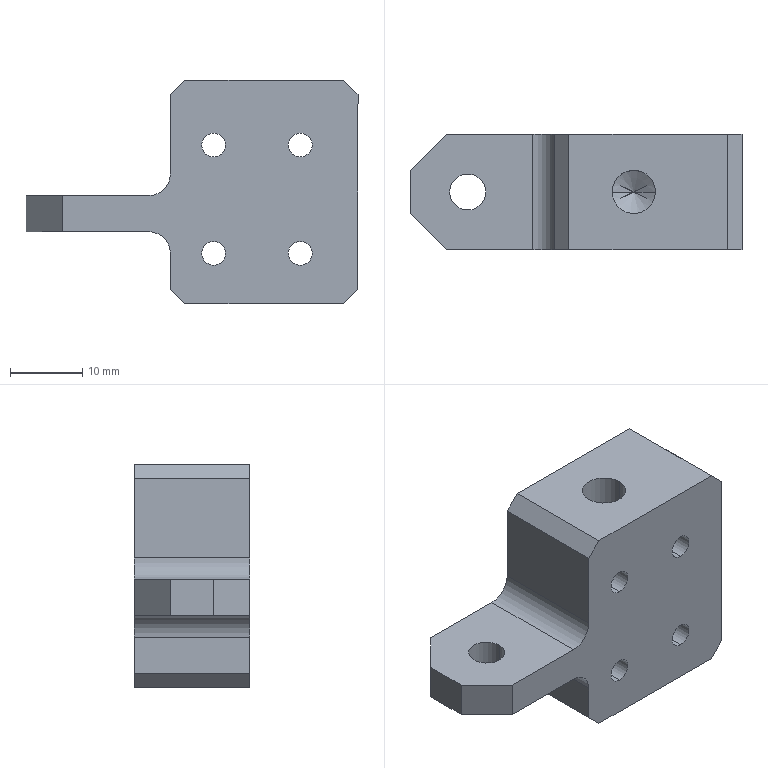Component | SolidWorks | XM-02-009A1-1 | 1 solid | 32 faces | box 46 x 16 x 31 mm | volume 13204 mm3 | plane 16 | cylinder 14 | cone 2 | commonest cylinder face diameters 3.3 x8 6 x4 5 x2 | material 45#
build123d program:
from build123d import *

# Parameters (mm, degrees)
SKETCH17_W            = 46
SKETCH17_H            = 5
BOSS_EXTRUDE1_DEPTH   = 16
SKETCH19_W            = 26
SKETCH19_H            = 16
BOSS_EXTRUDE2_DEPTH   = 16
M5_TAPPED_HOLE1_D     = 5
M6_TAPPED_HOLE1_D     = 6
M6_TAPPED_HOLE1_DEPTH = 15.5
M6_TAPPED_HOLE1_TIP   = 1.803
SKETCH30_W            = 26
SKETCH30_H            = 16
BOSS_EXTRUDE3_DEPTH   = 10
M4_TAPPED_HOLE2_D     = 3.3
CHAMFER1_SIZE         = 5
FILLET1_R             = 3
CHAMFER2_SIZE         = 2


with BuildPart() as part:
    # Sketch17 → Boss-Extrude1 (new body)
    with BuildSketch(Plane.XZ):
        with Locations((-23, 2.5)):
            Rectangle(SKETCH17_W, SKETCH17_H)
    extrude(amount=BOSS_EXTRUDE1_DEPTH)

    # Sketch19 → Boss-Extrude2 (add)
    with BuildSketch(Plane.XY.offset(5)):
        with Locations((-13, -8)):
            Rectangle(SKETCH19_W, SKETCH19_H)
    extrude(amount=BOSS_EXTRUDE2_DEPTH)

    # M5 Tapped Hole1 (through all)
    with Locations(Plane(origin=(0, 0, 0), x_dir=(-1, 0, 0), z_dir=(0, 0, -1))):
        with Locations((38, -8)):
            Hole(M5_TAPPED_HOLE1_D / 2)

    # M6 Tapped Hole1
    with Locations(Plane.XY.offset(21)):
        with Locations((-15, -8)):
            Hole(M6_TAPPED_HOLE1_D / 2, depth=M6_TAPPED_HOLE1_DEPTH)
            with Locations((0, 0, -(M6_TAPPED_HOLE1_DEPTH + M6_TAPPED_HOLE1_TIP / 2))):  # 118° drill point
                Cone(0, M6_TAPPED_HOLE1_D / 2, M6_TAPPED_HOLE1_TIP, mode=Mode.SUBTRACT)

    # Sketch30 → Boss-Extrude3 (add)
    with BuildSketch(Plane(origin=(0, 0, 0), x_dir=(-1, 0, 0), z_dir=(0, 0, -1))):
        with Locations((13, -8)):
            Rectangle(SKETCH30_W, SKETCH30_H)
    extrude(amount=BOSS_EXTRUDE3_DEPTH)

    # M4 Tapped Hole2 (through all)
    with Locations(Plane(origin=(0, 0, 0), x_dir=(1, 0, 0), z_dir=(0, 1, 0))):
        with Locations((-20, -12), (-8, -12), (-8, 3), (-20, 3)):
            Hole(M4_TAPPED_HOLE2_D / 2)

    # Chamfer1
    chamfer1_edges = [part.edges().sort_by_distance(p)[0] for p in [
        (-46, -16, 2.5),
        (-46, 0, 2.5),
    ]]
    chamfer(chamfer1_edges, length=CHAMFER1_SIZE)

    # Fillet1
    fillet1_edges = [part.edges().sort_by_distance(p)[0] for p in [
        (-26, -8, 5),
        (-26, -8, 0),
    ]]
    fillet(fillet1_edges, radius=FILLET1_R)

    # Chamfer2
    chamfer2_edges = [part.edges().sort_by_distance(p)[0] for p in [
        (-26, -8, 21),
        (0, -8, 21),
        (0, -8, -10),
        (-26, -8, -10),
    ]]
    chamfer(chamfer2_edges, length=CHAMFER2_SIZE)


solid = part.part

# Placed as in the assembly
solid = solid.moved(Location((-39, -3, -28), (0, 0, 0)))
STEP:
#1=COLOUR_RGB('',0.7922,0.8196,0.9333);
#2=FILL_AREA_STYLE_COLOUR('',#1);
#3=FILL_AREA_STYLE('',(#2));
#4=SURFACE_STYLE_FILL_AREA(#3);
#5=SURFACE_SIDE_STYLE('',(#4));
#6=SURFACE_STYLE_USAGE(.BOTH.,#5);
#7=PRESENTATION_STYLE_ASSIGNMENT((#6));
#8=CARTESIAN_POINT('',(-2.323,-0.748,-0.6949));
#9=VERTEX_POINT('',#8);
#10=CARTESIAN_POINT('',(-2.323,-0.748,-0.565));
#11=VERTEX_POINT('',#10);
#12=CARTESIAN_POINT('',(-2.323,-0.748,-0.6299));
#13=DIRECTION('',(0.,1.,0.));
#14=DIRECTION('',(0.,0.,1.));
#15=AXIS2_PLACEMENT_3D('',#12,#13,#14);
#16=CIRCLE('',#15,0.06496);
#17=EDGE_CURVE('',#9,#11,#16,.T.);
#18=ORIENTED_EDGE('',*,*,#17,.F.);
#19=CARTESIAN_POINT('',(-2.323,-0.1181,-0.6949));
#20=VERTEX_POINT('',#19);
#21=CARTESIAN_POINT('',(-2.323,-0.1181,-0.6949));
#22=DIRECTION('',(0.,1.,0.));
#23=VECTOR('',#22,39.37);
#24=LINE('',#21,#23);
#25=EDGE_CURVE('',#9,#20,#24,.T.);
#26=ORIENTED_EDGE('',*,*,#25,.T.);
#27=CARTESIAN_POINT('',(-2.323,-0.1181,-0.565));
#28=VERTEX_POINT('',#27);
#29=CARTESIAN_POINT('',(-2.323,-0.1181,-0.6299));
#30=DIRECTION('',(0.,1.,0.));
#31=DIRECTION('',(0.,0.,1.));
#32=AXIS2_PLACEMENT_3D('',#29,#30,#31);
#33=CIRCLE('',#32,0.06496);
#34=EDGE_CURVE('',#20,#28,#33,.T.);
#35=ORIENTED_EDGE('',*,*,#34,.T.);
#36=CARTESIAN_POINT('',(-2.323,-0.1181,-0.565));
#37=DIRECTION('',(0.,1.,0.));
#38=VECTOR('',#37,39.37);
#39=LINE('',#36,#38);
#40=EDGE_CURVE('',#11,#28,#39,.T.);
#41=ORIENTED_EDGE('',*,*,#40,.F.);
#42=EDGE_LOOP('',(#18,#26,#35,#41));
#43=FACE_OUTER_BOUND('',#42,.T.);
#44=CARTESIAN_POINT('',(-2.323,-0.1181,-0.6299));
#45=DIRECTION('',(0.,1.,0.));
#46=DIRECTION('',(0.,0.,1.));
#47=AXIS2_PLACEMENT_3D('',#44,#45,#46);
#48=CYLINDRICAL_SURFACE('',#47,0.06496);
#49=ADVANCED_FACE('',(#43),#48,.F.);
#50=CARTESIAN_POINT('',(-1.85,-0.748,-0.6949));
#51=VERTEX_POINT('',#50);
#52=CARTESIAN_POINT('',(-1.85,-0.748,-0.565));
#53=VERTEX_POINT('',#52);
#54=CARTESIAN_POINT('',(-1.85,-0.748,-0.6299));
#55=DIRECTION('',(0.,1.,0.));
#56=DIRECTION('',(0.,0.,1.));
#57=AXIS2_PLACEMENT_3D('',#54,#55,#56);
#58=CIRCLE('',#57,0.06496);
#59=EDGE_CURVE('',#51,#53,#58,.T.);
#60=ORIENTED_EDGE('',*,*,#59,.F.);
#61=CARTESIAN_POINT('',(-1.85,-0.1181,-0.6949));
#62=VERTEX_POINT('',#61);
#63=CARTESIAN_POINT('',(-1.85,-0.1181,-0.6949));
#64=DIRECTION('',(0.,1.,0.));
#65=VECTOR('',#64,39.37);
#66=LINE('',#63,#65);
#67=EDGE_CURVE('',#51,#62,#66,.T.);
#68=ORIENTED_EDGE('',*,*,#67,.T.);
#69=CARTESIAN_POINT('',(-1.85,-0.1181,-0.565));
#70=VERTEX_POINT('',#69);
#71=CARTESIAN_POINT('',(-1.85,-0.1181,-0.6299));
#72=DIRECTION('',(0.,1.,0.));
#73=DIRECTION('',(0.,0.,1.));
#74=AXIS2_PLACEMENT_3D('',#71,#72,#73);
#75=CIRCLE('',#74,0.06496);
#76=EDGE_CURVE('',#62,#70,#75,.T.);
#77=ORIENTED_EDGE('',*,*,#76,.T.);
#78=CARTESIAN_POINT('',(-1.85,-0.1181,-0.565));
#79=DIRECTION('',(0.,1.,0.));
#80=VECTOR('',#79,39.37);
#81=LINE('',#78,#80);
#82=EDGE_CURVE('',#53,#70,#81,.T.);
#83=ORIENTED_EDGE('',*,*,#82,.F.);
#84=EDGE_LOOP('',(#60,#68,#77,#83));
#85=FACE_OUTER_BOUND('',#84,.T.);
#86=CARTESIAN_POINT('',(-1.85,-0.1181,-0.6299));
#87=DIRECTION('',(0.,1.,0.));
#88=DIRECTION('',(0.,0.,1.));
#89=AXIS2_PLACEMENT_3D('',#86,#87,#88);
#90=CYLINDRICAL_SURFACE('',#89,0.06496);
#91=ADVANCED_FACE('',(#85),#90,.F.);
#92=CARTESIAN_POINT('',(-1.85,-0.748,-1.285));
#93=VERTEX_POINT('',#92);
#94=CARTESIAN_POINT('',(-1.85,-0.748,-1.156));
#95=VERTEX_POINT('',#94);
#96=CARTESIAN_POINT('',(-1.85,-0.748,-1.22));
#97=DIRECTION('',(0.,1.,0.));
#98=DIRECTION('',(0.,0.,1.));
#99=AXIS2_PLACEMENT_3D('',#96,#97,#98);
#100=CIRCLE('',#99,0.06496);
#101=EDGE_CURVE('',#93,#95,#100,.T.);
#102=ORIENTED_EDGE('',*,*,#101,.F.);
#103=CARTESIAN_POINT('',(-1.85,-0.1181,-1.285));
#104=VERTEX_POINT('',#103);
#105=CARTESIAN_POINT('',(-1.85,-0.1181,-1.285));
#106=DIRECTION('',(0.,1.,0.));
#107=VECTOR('',#106,39.37);
#108=LINE('',#105,#107);
#109=EDGE_CURVE('',#93,#104,#108,.T.);
#110=ORIENTED_EDGE('',*,*,#109,.T.);
#111=CARTESIAN_POINT('',(-1.85,-0.1181,-1.156));
#112=VERTEX_POINT('',#111);
#113=CARTESIAN_POINT('',(-1.85,-0.1181,-1.22));
#114=DIRECTION('',(0.,1.,0.));
#115=DIRECTION('',(0.,0.,1.));
#116=AXIS2_PLACEMENT_3D('',#113,#114,#115);
#117=CIRCLE('',#116,0.06496);
#118=EDGE_CURVE('',#104,#112,#117,.T.);
#119=ORIENTED_EDGE('',*,*,#118,.T.);
#120=CARTESIAN_POINT('',(-1.85,-0.1181,-1.156));
#121=DIRECTION('',(0.,1.,0.));
#122=VECTOR('',#121,39.37);
#123=LINE('',#120,#122);
#124=EDGE_CURVE('',#95,#112,#123,.T.);
#125=ORIENTED_EDGE('',*,*,#124,.F.);
#126=EDGE_LOOP('',(#102,#110,#119,#125));
#127=FACE_OUTER_BOUND('',#126,.T.);
#128=CARTESIAN_POINT('',(-1.85,-0.1181,-1.22));
#129=DIRECTION('',(0.,1.,0.));
#130=DIRECTION('',(0.,0.,1.));
#131=AXIS2_PLACEMENT_3D('',#128,#129,#130);
#132=CYLINDRICAL_SURFACE('',#131,0.06496);
#133=ADVANCED_FACE('',(#127),#132,.F.);
#134=CARTESIAN_POINT('',(-2.323,-0.748,-1.285));
#135=VERTEX_POINT('',#134);
#136=CARTESIAN_POINT('',(-2.323,-0.748,-1.156));
#137=VERTEX_POINT('',#136);
#138=CARTESIAN_POINT('',(-2.323,-0.748,-1.22));
#139=DIRECTION('',(0.,1.,0.));
#140=DIRECTION('',(0.,0.,1.));
#141=AXIS2_PLACEMENT_3D('',#138,#139,#140);
#142=CIRCLE('',#141,0.06496);
#143=EDGE_CURVE('',#135,#137,#142,.T.);
#144=ORIENTED_EDGE('',*,*,#143,.F.);
#145=CARTESIAN_POINT('',(-2.323,-0.1181,-1.285));
#146=VERTEX_POINT('',#145);
#147=CARTESIAN_POINT('',(-2.323,-0.1181,-1.285));
#148=DIRECTION('',(0.,1.,0.));
#149=VECTOR('',#148,39.37);
#150=LINE('',#147,#149);
#151=EDGE_CURVE('',#135,#146,#150,.T.);
#152=ORIENTED_EDGE('',*,*,#151,.T.);
#153=CARTESIAN_POINT('',(-2.323,-0.1181,-1.156));
#154=VERTEX_POINT('',#153);
#155=CARTESIAN_POINT('',(-2.323,-0.1181,-1.22));
#156=DIRECTION('',(0.,1.,0.));
#157=DIRECTION('',(0.,0.,1.));
#158=AXIS2_PLACEMENT_3D('',#155,#156,#157);
#159=CIRCLE('',#158,0.06496);
#160=EDGE_CURVE('',#146,#154,#159,.T.);
#161=ORIENTED_EDGE('',*,*,#160,.T.);
#162=CARTESIAN_POINT('',(-2.323,-0.1181,-1.156));
#163=DIRECTION('',(0.,1.,0.));
#164=VECTOR('',#163,39.37);
#165=LINE('',#162,#164);
#166=EDGE_CURVE('',#137,#154,#165,.T.);
#167=ORIENTED_EDGE('',*,*,#166,.F.);
#168=EDGE_LOOP('',(#144,#152,#161,#167));
#169=FACE_OUTER_BOUND('',#168,.T.);
#170=CARTESIAN_POINT('',(-2.323,-0.1181,-1.22));
#171=DIRECTION('',(0.,1.,0.));
#172=DIRECTION('',(0.,0.,1.));
#173=AXIS2_PLACEMENT_3D('',#170,#171,#172);
#174=CYLINDRICAL_SURFACE('',#173,0.06496);
#175=ADVANCED_FACE('',(#169),#174,.F.);
#176=CARTESIAN_POINT('',(-2.244,-0.4331,-0.8858));
#177=VERTEX_POINT('',#176);
#178=CARTESIAN_POINT('',(-2.008,-0.4331,-0.8858));
#179=VERTEX_POINT('',#178);
#180=CARTESIAN_POINT('',(-2.126,-0.4331,-0.8858));
#181=DIRECTION('',(0.,0.,1.));
#182=DIRECTION('',(1.,0.,0.));
#183=AXIS2_PLACEMENT_3D('',#180,#181,#182);
#184=CIRCLE('',#183,0.1181);
#185=EDGE_CURVE('',#177,#179,#184,.T.);
#186=ORIENTED_EDGE('',*,*,#185,.F.);
#187=CARTESIAN_POINT('',(-2.244,-0.4331,-0.2756));
#188=VERTEX_POINT('',#187);
#189=CARTESIAN_POINT('',(-2.244,-0.4331,-0.2756));
#190=DIRECTION('',(0.,0.,1.));
#191=VECTOR('',#190,39.37);
#192=LINE('',#189,#191);
#193=EDGE_CURVE('',#177,#188,#192,.T.);
#194=ORIENTED_EDGE('',*,*,#193,.T.);
#195=CARTESIAN_POINT('',(-2.008,-0.4331,-0.2756));
#196=VERTEX_POINT('',#195);
#197=CARTESIAN_POINT('',(-2.126,-0.4331,-0.2756));
#198=DIRECTION('',(0.,0.,1.));
#199=DIRECTION('',(1.,0.,0.));
#200=AXIS2_PLACEMENT_3D('',#197,#198,#199);
#201=CIRCLE('',#200,0.1181);
#202=EDGE_CURVE('',#188,#196,#201,.T.);
#203=ORIENTED_EDGE('',*,*,#202,.T.);
#204=CARTESIAN_POINT('',(-2.008,-0.4331,-0.2756));
#205=DIRECTION('',(0.,0.,1.));
#206=VECTOR('',#205,39.37);
#207=LINE('',#204,#206);
#208=EDGE_CURVE('',#179,#196,#207,.T.);
#209=ORIENTED_EDGE('',*,*,#208,.F.);
#210=EDGE_LOOP('',(#186,#194,#203,#209));
#211=FACE_OUTER_BOUND('',#210,.T.);
#212=CARTESIAN_POINT('',(-2.126,-0.4331,-0.2756));
#213=DIRECTION('',(0.,0.,1.));
#214=DIRECTION('',(1.,0.,0.));
#215=AXIS2_PLACEMENT_3D('',#212,#213,#214);
#216=CYLINDRICAL_SURFACE('',#215,0.1181);
#217=ADVANCED_FACE('',(#211),#216,.F.);
#218=CARTESIAN_POINT('',(-2.126,-0.4331,-0.9568));
#219=VERTEX_POINT('',#218);
#220=CARTESIAN_POINT('',(-2.008,-0.4331,-0.8858));
#221=DIRECTION('',(0.8572,0.,0.515));
#222=VECTOR('',#221,39.37);
#223=LINE('',#220,#222);
#224=EDGE_CURVE('',#219,#179,#223,.T.);
#225=ORIENTED_EDGE('',*,*,#224,.F.);
#226=CARTESIAN_POINT('',(-2.244,-0.4331,-0.8858));
#227=DIRECTION('',(-0.8572,0.,0.515));
#228=VECTOR('',#227,39.37);
#229=LINE('',#226,#228);
#230=EDGE_CURVE('',#219,#177,#229,.T.);
#231=ORIENTED_EDGE('',*,*,#230,.T.);
#232=ORIENTED_EDGE('',*,*,#185,.T.);
#233=EDGE_LOOP('',(#225,#231,#232));
#234=FACE_OUTER_BOUND('',#233,.T.);
#235=CARTESIAN_POINT('',(-2.126,-0.4331,-0.8858));
#236=DIRECTION('',(0.,0.,1.));
#237=DIRECTION('',(1.,0.,0.));
#238=AXIS2_PLACEMENT_3D('',#235,#236,#237);
#239=CONICAL_SURFACE('',#238,0.1181,1.03);
#240=ADVANCED_FACE('',(#234),#239,.F.);
#241=CARTESIAN_POINT('',(-3.13,-0.4331,-0.9055));
#242=VERTEX_POINT('',#241);
#243=CARTESIAN_POINT('',(-2.933,-0.4331,-0.9055));
#244=VERTEX_POINT('',#243);
#245=CARTESIAN_POINT('',(-3.031,-0.4331,-0.9055));
#246=DIRECTION('',(-0.,0.,1.));
#247=DIRECTION('',(-1.,0.,0.));
#248=AXIS2_PLACEMENT_3D('',#245,#246,#247);
#249=CIRCLE('',#248,0.09843);
#250=EDGE_CURVE('',#242,#244,#249,.T.);
#251=ORIENTED_EDGE('',*,*,#250,.T.);
#252=CARTESIAN_POINT('',(-2.933,-0.4331,-1.102));
#253=VERTEX_POINT('',#252);
#254=CARTESIAN_POINT('',(-2.933,-0.4331,-1.102));
#255=DIRECTION('',(0.,0.,-1.));
#256=VECTOR('',#255,39.37);
#257=LINE('',#254,#256);
#258=EDGE_CURVE('',#244,#253,#257,.T.);
#259=ORIENTED_EDGE('',*,*,#258,.T.);
#260=CARTESIAN_POINT('',(-3.13,-0.4331,-1.102));
#261=VERTEX_POINT('',#260);
#262=CARTESIAN_POINT('',(-3.031,-0.4331,-1.102));
#263=DIRECTION('',(0.,0.,-1.));
#264=DIRECTION('',(-1.,0.,0.));
#265=AXIS2_PLACEMENT_3D('',#262,#263,#264);
#266=CIRCLE('',#265,0.09843);
#267=EDGE_CURVE('',#253,#261,#266,.T.);
#268=ORIENTED_EDGE('',*,*,#267,.T.);
#269=CARTESIAN_POINT('',(-3.13,-0.4331,-1.102));
#270=DIRECTION('',(0.,0.,-1.));
#271=VECTOR('',#270,39.37);
#272=LINE('',#269,#271);
#273=EDGE_CURVE('',#242,#261,#272,.T.);
#274=ORIENTED_EDGE('',*,*,#273,.F.);
#275=EDGE_LOOP('',(#251,#259,#268,#274));
#276=FACE_OUTER_BOUND('',#275,.T.);
#277=CARTESIAN_POINT('',(-3.031,-0.4331,-1.102));
#278=DIRECTION('',(0.,0.,-1.));
#279=DIRECTION('',(-1.,0.,0.));
#280=AXIS2_PLACEMENT_3D('',#277,#278,#279);
#281=CYLINDRICAL_SURFACE('',#280,0.09843);
#282=ADVANCED_FACE('',(#276),#281,.F.);
#283=CARTESIAN_POINT('',(-1.535,-0.748,-1.417));
#284=VERTEX_POINT('',#283);
#285=CARTESIAN_POINT('',(-1.535,-0.748,-0.3543));
#286=VERTEX_POINT('',#285);
#287=CARTESIAN_POINT('',(-1.535,-0.748,-1.102));
#288=DIRECTION('',(0.,0.,1.));
#289=VECTOR('',#288,39.37);
#290=LINE('',#287,#289);
#291=EDGE_CURVE('',#284,#286,#290,.T.);
#292=ORIENTED_EDGE('',*,*,#291,.T.);
#293=CARTESIAN_POINT('',(-1.614,-0.748,-0.2756));
#294=VERTEX_POINT('',#293);
#295=CARTESIAN_POINT('',(-1.161,-0.748,-0.7283));
#296=DIRECTION('',(-0.7071,0.,0.7071));
#297=VECTOR('',#296,39.37);
#298=LINE('',#295,#297);
#299=EDGE_CURVE('',#286,#294,#298,.T.);
#300=ORIENTED_EDGE('',*,*,#299,.T.);
#301=CARTESIAN_POINT('',(-2.48,-0.748,-0.2756));
#302=VERTEX_POINT('',#301);
#303=CARTESIAN_POINT('',(-2.559,-0.748,-0.2756));
#304=DIRECTION('',(1.,0.,0.));
#305=VECTOR('',#304,39.37);
#306=LINE('',#303,#305);
#307=EDGE_CURVE('',#302,#294,#306,.T.);
#308=ORIENTED_EDGE('',*,*,#307,.F.);
#309=CARTESIAN_POINT('',(-2.559,-0.748,-0.3543));
#310=VERTEX_POINT('',#309);
#311=CARTESIAN_POINT('',(-2.421,-0.748,-0.2165));
#312=DIRECTION('',(-0.7071,0.,-0.7071));
#313=VECTOR('',#312,39.37);
#314=LINE('',#311,#313);
#315=EDGE_CURVE('',#302,#310,#314,.T.);
#316=ORIENTED_EDGE('',*,*,#315,.T.);
#317=CARTESIAN_POINT('',(-2.559,-0.748,-0.7874));
#318=VERTEX_POINT('',#317);
#319=CARTESIAN_POINT('',(-2.559,-0.748,-0.2756));
#320=DIRECTION('',(0.,0.,-1.));
#321=VECTOR('',#320,39.37);
#322=LINE('',#319,#321);
#323=EDGE_CURVE('',#310,#318,#322,.T.);
#324=ORIENTED_EDGE('',*,*,#323,.T.);
#325=CARTESIAN_POINT('',(-2.677,-0.748,-0.9055));
#326=VERTEX_POINT('',#325);
#327=CARTESIAN_POINT('',(-2.677,-0.748,-0.7874));
#328=DIRECTION('',(0.,1.,0.));
#329=DIRECTION('',(0.,0.,-1.));
#330=AXIS2_PLACEMENT_3D('',#327,#328,#329);
#331=CIRCLE('',#330,0.1181);
#332=EDGE_CURVE('',#318,#326,#331,.T.);
#333=ORIENTED_EDGE('',*,*,#332,.T.);
#334=CARTESIAN_POINT('',(-3.15,-0.748,-0.9055));
#335=VERTEX_POINT('',#334);
#336=CARTESIAN_POINT('',(-1.535,-0.748,-0.9055));
#337=DIRECTION('',(-1.,0.,-0.));
#338=VECTOR('',#337,39.37);
#339=LINE('',#336,#338);
#340=EDGE_CURVE('',#326,#335,#339,.T.);
#341=ORIENTED_EDGE('',*,*,#340,.T.);
#342=CARTESIAN_POINT('',(-3.15,-0.748,-1.102));
#343=VERTEX_POINT('',#342);
#344=CARTESIAN_POINT('',(-3.15,-0.748,-1.102));
#345=DIRECTION('',(0.,0.,-1.));
#346=VECTOR('',#345,39.37);
#347=LINE('',#344,#346);
#348=EDGE_CURVE('',#335,#343,#347,.T.);
#349=ORIENTED_EDGE('',*,*,#348,.T.);
#350=CARTESIAN_POINT('',(-2.677,-0.748,-1.102));
#351=VERTEX_POINT('',#350);
#352=CARTESIAN_POINT('',(-1.535,-0.748,-1.102));
#353=DIRECTION('',(-1.,0.,-0.));
#354=VECTOR('',#353,39.37);
#355=LINE('',#352,#354);
#356=EDGE_CURVE('',#351,#343,#355,.T.);
#357=ORIENTED_EDGE('',*,*,#356,.F.);
#358=CARTESIAN_POINT('',(-2.559,-0.748,-1.22));
#359=VERTEX_POINT('',#358);
#360=CARTESIAN_POINT('',(-2.677,-0.748,-1.22));
#361=DIRECTION('',(0.,1.,0.));
#362=DIRECTION('',(0.,0.,-1.));
#363=AXIS2_PLACEMENT_3D('',#360,#361,#362);
#364=CIRCLE('',#363,0.1181);
#365=EDGE_CURVE('',#351,#359,#364,.T.);
#366=ORIENTED_EDGE('',*,*,#365,.T.);
#367=CARTESIAN_POINT('',(-2.559,-0.748,-1.417));
#368=VERTEX_POINT('',#367);
#369=CARTESIAN_POINT('',(-2.559,-0.748,-1.496));
#370=DIRECTION('',(-0.,0.,1.));
#371=VECTOR('',#370,39.37);
#372=LINE('',#369,#371);
#373=EDGE_CURVE('',#368,#359,#372,.T.);
#374=ORIENTED_EDGE('',*,*,#373,.F.);
#375=CARTESIAN_POINT('',(-2.48,-0.748,-1.496));
#376=VERTEX_POINT('',#375);
#377=CARTESIAN_POINT('',(-2.205,-0.748,-1.772));
#378=DIRECTION('',(0.7071,0.,-0.7071));
#379=VECTOR('',#378,39.37);
#380=LINE('',#377,#379);
#381=EDGE_CURVE('',#368,#376,#380,.T.);
#382=ORIENTED_EDGE('',*,*,#381,.T.);
#383=CARTESIAN_POINT('',(-1.614,-0.748,-1.496));
#384=VERTEX_POINT('',#383);
#385=CARTESIAN_POINT('',(-1.535,-0.748,-1.496));
#386=DIRECTION('',(-1.,0.,-0.));
#387=VECTOR('',#386,39.37);
#388=LINE('',#385,#387);
#389=EDGE_CURVE('',#384,#376,#388,.T.);
#390=ORIENTED_EDGE('',*,*,#389,.F.);
#391=CARTESIAN_POINT('',(-1.378,-0.748,-1.26));
#392=DIRECTION('',(0.7071,0.,0.7071));
#393=VECTOR('',#392,39.37);
#394=LINE('',#391,#393);
#395=EDGE_CURVE('',#384,#284,#394,.T.);
#396=ORIENTED_EDGE('',*,*,#395,.T.);
#397=EDGE_LOOP('',(#292,#300,#308,#316,#324,#333,#341,#349,#357,#366,#374,#382,#390,#396));
#398=FACE_OUTER_BOUND('',#397,.T.);
#399=CARTESIAN_POINT('',(-2.323,-0.748,-1.22));
#400=DIRECTION('',(0.,1.,0.));
#401=DIRECTION('',(0.,0.,1.));
#402=AXIS2_PLACEMENT_3D('',#399,#400,#401);
#403=CIRCLE('',#402,0.06496);
#404=EDGE_CURVE('',#137,#135,#403,.T.);
#405=ORIENTED_EDGE('',*,*,#404,.T.);
#406=ORIENTED_EDGE('',*,*,#143,.T.);
#407=EDGE_LOOP('',(#405,#406));
#408=FACE_BOUND('',#407,.T.);
#409=CARTESIAN_POINT('',(-1.85,-0.748,-1.22));
#410=DIRECTION('',(0.,1.,0.));
#411=DIRECTION('',(0.,0.,1.));
#412=AXIS2_PLACEMENT_3D('',#409,#410,#411);
#413=CIRCLE('',#412,0.06496);
#414=EDGE_CURVE('',#95,#93,#413,.T.);
#415=ORIENTED_EDGE('',*,*,#414,.T.);
#416=ORIENTED_EDGE('',*,*,#101,.T.);
#417=EDGE_LOOP('',(#415,#416));
#418=FACE_BOUND('',#417,.T.);
#419=CARTESIAN_POINT('',(-1.85,-0.748,-0.6299));
#420=DIRECTION('',(0.,1.,0.));
#421=DIRECTION('',(0.,0.,1.));
#422=AXIS2_PLACEMENT_3D('',#419,#420,#421);
#423=CIRCLE('',#422,0.06496);
#424=EDGE_CURVE('',#53,#51,#423,.T.);
#425=ORIENTED_EDGE('',*,*,#424,.T.);
#426=ORIENTED_EDGE('',*,*,#59,.T.);
#427=EDGE_LOOP('',(#425,#426));
#428=FACE_BOUND('',#427,.T.);
#429=CARTESIAN_POINT('',(-2.323,-0.748,-0.6299));
#430=DIRECTION('',(0.,1.,0.));
#431=DIRECTION('',(0.,0.,1.));
#432=AXIS2_PLACEMENT_3D('',#429,#430,#431);
#433=CIRCLE('',#432,0.06496);
#434=EDGE_CURVE('',#11,#9,#433,.T.);
#435=ORIENTED_EDGE('',*,*,#434,.T.);
#436=ORIENTED_EDGE('',*,*,#17,.T.);
#437=EDGE_LOOP('',(#435,#436));
#438=FACE_BOUND('',#437,.T.);
#439=CARTESIAN_POINT('',(-1.535,-0.748,-1.102));
#440=DIRECTION('',(0.,-1.,0.));
#441=DIRECTION('',(0.,0.,-1.));
#442=AXIS2_PLACEMENT_3D('',#439,#440,#441);
#443=PLANE('',#442);
#444=ADVANCED_FACE('',(#398,#408,#418,#428,#438),#443,.T.);
#445=CARTESIAN_POINT('',(-2.323,-0.1181,-0.6299));
#446=DIRECTION('',(0.,1.,0.));
#447=DIRECTION('',(0.,0.,1.));
#448=AXIS2_PLACEMENT_3D('',#445,#446,#447);
#449=CIRCLE('',#448,0.06496);
#450=EDGE_CURVE('',#28,#20,#449,.T.);
#451=ORIENTED_EDGE('',*,*,#450,.F.);
#452=ORIENTED_EDGE('',*,*,#34,.F.);
#453=EDGE_LOOP('',(#451,#452));
#454=FACE_BOUND('',#453,.T.);
#455=CARTESIAN_POINT('',(-1.85,-0.1181,-1.22));
#456=DIRECTION('',(0.,1.,0.));
#457=DIRECTION('',(0.,0.,1.));
#458=AXIS2_PLACEMENT_3D('',#455,#456,#457);
#459=CIRCLE('',#458,0.06496);
#460=EDGE_CURVE('',#112,#104,#459,.T.);
#461=ORIENTED_EDGE('',*,*,#460,.F.);
#462=ORIENTED_EDGE('',*,*,#118,.F.);
#463=EDGE_LOOP('',(#461,#462));
#464=FACE_BOUND('',#463,.T.);
#465=CARTESIAN_POINT('',(-2.323,-0.1181,-1.22));
#466=DIRECTION('',(0.,1.,0.));
#467=DIRECTION('',(0.,0.,1.));
#468=AXIS2_PLACEMENT_3D('',#465,#466,#467);
#469=CIRCLE('',#468,0.06496);
#470=EDGE_CURVE('',#154,#146,#469,.T.);
#471=ORIENTED_EDGE('',*,*,#470,.F.);
#472=ORIENTED_EDGE('',*,*,#160,.F.);
#473=EDGE_LOOP('',(#471,#472));
#474=FACE_BOUND('',#473,.T.);
#475=CARTESIAN_POINT('',(-1.614,-0.1181,-0.2756));
#476=VERTEX_POINT('',#475);
#477=CARTESIAN_POINT('',(-2.48,-0.1181,-0.2756));
#478=VERTEX_POINT('',#477);
#479=CARTESIAN_POINT('',(-2.559,-0.1181,-0.2756));
#480=DIRECTION('',(-1.,0.,0.));
#481=VECTOR('',#480,39.37);
#482=LINE('',#479,#481);
#483=EDGE_CURVE('',#476,#478,#482,.T.);
#484=ORIENTED_EDGE('',*,*,#483,.F.);
#485=CARTESIAN_POINT('',(-1.535,-0.1181,-0.3543));
#486=VERTEX_POINT('',#485);
#487=CARTESIAN_POINT('',(-1.614,-0.1181,-0.2756));
#488=DIRECTION('',(0.7071,0.,-0.7071));
#489=VECTOR('',#488,39.37);
#490=LINE('',#487,#489);
#491=EDGE_CURVE('',#476,#486,#490,.T.);
#492=ORIENTED_EDGE('',*,*,#491,.T.);
#493=CARTESIAN_POINT('',(-1.535,-0.1181,-1.417));
#494=VERTEX_POINT('',#493);
#495=CARTESIAN_POINT('',(-1.535,-0.1181,-1.102));
#496=DIRECTION('',(0.,0.,1.));
#497=VECTOR('',#496,39.37);
#498=LINE('',#495,#497);
#499=EDGE_CURVE('',#494,#486,#498,.T.);
#500=ORIENTED_EDGE('',*,*,#499,.F.);
#501=CARTESIAN_POINT('',(-1.614,-0.1181,-1.496));
#502=VERTEX_POINT('',#501);
#503=CARTESIAN_POINT('',(-1.614,-0.1181,-1.496));
#504=DIRECTION('',(-0.7071,0.,-0.7071));
#505=VECTOR('',#504,39.37);
#506=LINE('',#503,#505);
#507=EDGE_CURVE('',#494,#502,#506,.T.);
#508=ORIENTED_EDGE('',*,*,#507,.T.);
#509=CARTESIAN_POINT('',(-2.48,-0.1181,-1.496));
#510=VERTEX_POINT('',#509);
#511=CARTESIAN_POINT('',(-1.535,-0.1181,-1.496));
#512=DIRECTION('',(1.,0.,0.));
#513=VECTOR('',#512,39.37);
#514=LINE('',#511,#513);
#515=EDGE_CURVE('',#510,#502,#514,.T.);
#516=ORIENTED_EDGE('',*,*,#515,.F.);
#517=CARTESIAN_POINT('',(-2.559,-0.1181,-1.417));
#518=VERTEX_POINT('',#517);
#519=CARTESIAN_POINT('',(-2.48,-0.1181,-1.496));
#520=DIRECTION('',(-0.7071,0.,0.7071));
#521=VECTOR('',#520,39.37);
#522=LINE('',#519,#521);
#523=EDGE_CURVE('',#510,#518,#522,.T.);
#524=ORIENTED_EDGE('',*,*,#523,.T.);
#525=CARTESIAN_POINT('',(-2.559,-0.1181,-1.22));
#526=VERTEX_POINT('',#525);
#527=CARTESIAN_POINT('',(-2.559,-0.1181,-1.496));
#528=DIRECTION('',(-0.,0.,1.));
#529=VECTOR('',#528,39.37);
#530=LINE('',#527,#529);
#531=EDGE_CURVE('',#518,#526,#530,.T.);
#532=ORIENTED_EDGE('',*,*,#531,.T.);
#533=CARTESIAN_POINT('',(-2.677,-0.1181,-1.102));
#534=VERTEX_POINT('',#533);
#535=CARTESIAN_POINT('',(-2.677,-0.1181,-1.22));
#536=DIRECTION('',(0.,-1.,0.));
#537=DIRECTION('',(0.,0.,-1.));
#538=AXIS2_PLACEMENT_3D('',#535,#536,#537);
#539=CIRCLE('',#538,0.1181);
#540=EDGE_CURVE('',#526,#534,#539,.T.);
#541=ORIENTED_EDGE('',*,*,#540,.T.);
#542=CARTESIAN_POINT('',(-3.15,-0.1181,-1.102));
#543=VERTEX_POINT('',#542);
#544=CARTESIAN_POINT('',(-1.535,-0.1181,-1.102));
#545=DIRECTION('',(-1.,0.,-0.));
#546=VECTOR('',#545,39.37);
#547=LINE('',#544,#546);
#548=EDGE_CURVE('',#534,#543,#547,.T.);
#549=ORIENTED_EDGE('',*,*,#548,.T.);
#550=CARTESIAN_POINT('',(-3.15,-0.1181,-0.9055));
#551=VERTEX_POINT('',#550);
#552=CARTESIAN_POINT('',(-3.15,-0.1181,-0.9055));
#553=DIRECTION('',(0.,0.,1.));
#554=VECTOR('',#553,39.37);
#555=LINE('',#552,#554);
#556=EDGE_CURVE('',#543,#551,#555,.T.);
#557=ORIENTED_EDGE('',*,*,#556,.T.);
#558=CARTESIAN_POINT('',(-2.677,-0.1181,-0.9055));
#559=VERTEX_POINT('',#558);
#560=CARTESIAN_POINT('',(-1.535,-0.1181,-0.9055));
#561=DIRECTION('',(-1.,0.,-0.));
#562=VECTOR('',#561,39.37);
#563=LINE('',#560,#562);
#564=EDGE_CURVE('',#559,#551,#563,.T.);
#565=ORIENTED_EDGE('',*,*,#564,.F.);
#566=CARTESIAN_POINT('',(-2.559,-0.1181,-0.7874));
#567=VERTEX_POINT('',#566);
#568=CARTESIAN_POINT('',(-2.677,-0.1181,-0.7874));
#569=DIRECTION('',(0.,-1.,0.));
#570=DIRECTION('',(0.,0.,-1.));
#571=AXIS2_PLACEMENT_3D('',#568,#569,#570);
#572=CIRCLE('',#571,0.1181);
#573=EDGE_CURVE('',#559,#567,#572,.T.);
#574=ORIENTED_EDGE('',*,*,#573,.T.);
#575=CARTESIAN_POINT('',(-2.559,-0.1181,-0.3543));
#576=VERTEX_POINT('',#575);
#577=CARTESIAN_POINT('',(-2.559,-0.1181,-0.2756));
#578=DIRECTION('',(0.,0.,-1.));
#579=VECTOR('',#578,39.37);
#580=LINE('',#577,#579);
#581=EDGE_CURVE('',#576,#567,#580,.T.);
#582=ORIENTED_EDGE('',*,*,#581,.F.);
#583=CARTESIAN_POINT('',(-2.48,-0.1181,-0.2756));
#584=DIRECTION('',(0.7071,0.,0.7071));
#585=VECTOR('',#584,39.37);
#586=LINE('',#583,#585);
#587=EDGE_CURVE('',#576,#478,#586,.T.);
#588=ORIENTED_EDGE('',*,*,#587,.T.);
#589=EDGE_LOOP('',(#484,#492,#500,#508,#516,#524,#532,#541,#549,#557,#565,#574,#582,#588));
#590=FACE_OUTER_BOUND('',#589,.T.);
#591=CARTESIAN_POINT('',(-1.85,-0.1181,-0.6299));
#592=DIRECTION('',(0.,1.,0.));
#593=DIRECTION('',(0.,0.,1.));
#594=AXIS2_PLACEMENT_3D('',#591,#592,#593);
#595=CIRCLE('',#594,0.06496);
#596=EDGE_CURVE('',#70,#62,#595,.T.);
#597=ORIENTED_EDGE('',*,*,#596,.F.);
#598=ORIENTED_EDGE('',*,*,#76,.F.);
#599=EDGE_LOOP('',(#597,#598));
#600=FACE_BOUND('',#599,.T.);
#601=CARTESIAN_POINT('',(-1.535,-0.1181,-1.102));
#602=DIRECTION('',(0.,-1.,0.));
#603=DIRECTION('',(0.,0.,-1.));
#604=AXIS2_PLACEMENT_3D('',#601,#602,#603);
#605=PLANE('',#604);
#606=ADVANCED_FACE('',(#454,#464,#474,#590,#600),#605,.F.);
#607=ORIENTED_EDGE('',*,*,#340,.F.);
#608=CARTESIAN_POINT('',(-2.677,-0.1181,-0.9055));
#609=DIRECTION('',(-0.,1.,-0.));
#610=VECTOR('',#609,39.37);
#611=LINE('',#608,#610);
#612=EDGE_CURVE('',#326,#559,#611,.T.);
#613=ORIENTED_EDGE('',*,*,#612,.T.);
#614=ORIENTED_EDGE('',*,*,#564,.T.);
#615=CARTESIAN_POINT('',(-3.346,-0.315,-0.9055));
#616=VERTEX_POINT('',#615);
#617=CARTESIAN_POINT('',(-3.15,-0.1181,-0.9055));
#618=DIRECTION('',(-0.7071,-0.7071,-0.));
#619=VECTOR('',#618,39.37);
#620=LINE('',#617,#619);
#621=EDGE_CURVE('',#551,#616,#620,.T.);
#622=ORIENTED_EDGE('',*,*,#621,.T.);
#623=CARTESIAN_POINT('',(-3.346,-0.5512,-0.9055));
#624=VERTEX_POINT('',#623);
#625=CARTESIAN_POINT('',(-3.346,-0.748,-0.9055));
#626=DIRECTION('',(0.,1.,0.));
#627=VECTOR('',#626,39.37);
#628=LINE('',#625,#627);
#629=EDGE_CURVE('',#624,#616,#628,.T.);
#630=ORIENTED_EDGE('',*,*,#629,.F.);
#631=CARTESIAN_POINT('',(-3.346,-0.5512,-0.9055));
#632=DIRECTION('',(0.7071,-0.7071,0.));
#633=VECTOR('',#632,39.37);
#634=LINE('',#631,#633);
#635=EDGE_CURVE('',#624,#335,#634,.T.);
#636=ORIENTED_EDGE('',*,*,#635,.T.);
#637=EDGE_LOOP('',(#607,#613,#614,#622,#630,#636));
#638=FACE_OUTER_BOUND('',#637,.T.);
#639=ORIENTED_EDGE('',*,*,#250,.F.);
#640=CARTESIAN_POINT('',(-3.031,-0.4331,-0.9055));
#641=DIRECTION('',(-0.,0.,1.));
#642=DIRECTION('',(-1.,0.,0.));
#643=AXIS2_PLACEMENT_3D('',#640,#641,#642);
#644=CIRCLE('',#643,0.09843);
#645=EDGE_CURVE('',#244,#242,#644,.T.);
#646=ORIENTED_EDGE('',*,*,#645,.F.);
#647=EDGE_LOOP('',(#639,#646));
#648=FACE_BOUND('',#647,.T.);
#649=CARTESIAN_POINT('',(-1.535,-0.748,-0.9055));
#650=DIRECTION('',(0.,0.,-1.));
#651=DIRECTION('',(-1.,0.,-0.));
#652=AXIS2_PLACEMENT_3D('',#649,#650,#651);
#653=PLANE('',#652);
#654=ADVANCED_FACE('',(#638,#648),#653,.F.);
#655=ORIENTED_EDGE('',*,*,#499,.T.);
#656=CARTESIAN_POINT('',(-1.535,-0.748,-0.3543));
#657=DIRECTION('',(0.,-1.,0.));
#658=VECTOR('',#657,39.37);
#659=LINE('',#656,#658);
#660=EDGE_CURVE('',#486,#286,#659,.T.);
#661=ORIENTED_EDGE('',*,*,#660,.T.);
#662=ORIENTED_EDGE('',*,*,#291,.F.);
#663=CARTESIAN_POINT('',(-1.535,-0.1181,-1.417));
#664=DIRECTION('',(0.,1.,0.));
#665=VECTOR('',#664,39.37);
#666=LINE('',#663,#665);
#667=EDGE_CURVE('',#284,#494,#666,.T.);
#668=ORIENTED_EDGE('',*,*,#667,.T.);
#669=EDGE_LOOP('',(#655,#661,#662,#668));
#670=FACE_OUTER_BOUND('',#669,.T.);
#671=CARTESIAN_POINT('',(-1.535,-0.748,-1.102));
#672=DIRECTION('',(-1.,0.,0.));
#673=DIRECTION('',(0.,0.,1.));
#674=AXIS2_PLACEMENT_3D('',#671,#672,#673);
#675=PLANE('',#674);
#676=ADVANCED_FACE('',(#670),#675,.F.);
#677=ORIENTED_EDGE('',*,*,#629,.T.);
#678=CARTESIAN_POINT('',(-3.346,-0.315,-1.102));
#679=VERTEX_POINT('',#678);
#680=CARTESIAN_POINT('',(-3.346,-0.315,-1.102));
#681=DIRECTION('',(0.,0.,-1.));
#682=VECTOR('',#681,39.37);
#683=LINE('',#680,#682);
#684=EDGE_CURVE('',#616,#679,#683,.T.);
#685=ORIENTED_EDGE('',*,*,#684,.T.);
#686=CARTESIAN_POINT('',(-3.346,-0.5512,-1.102));
#687=VERTEX_POINT('',#686);
#688=CARTESIAN_POINT('',(-3.346,-0.748,-1.102));
#689=DIRECTION('',(0.,1.,0.));
#690=VECTOR('',#689,39.37);
#691=LINE('',#688,#690);
#692=EDGE_CURVE('',#687,#679,#691,.T.);
#693=ORIENTED_EDGE('',*,*,#692,.F.);
#694=CARTESIAN_POINT('',(-3.346,-0.5512,-1.102));
#695=DIRECTION('',(0.,0.,1.));
#696=VECTOR('',#695,39.37);
#697=LINE('',#694,#696);
#698=EDGE_CURVE('',#687,#624,#697,.T.);
#699=ORIENTED_EDGE('',*,*,#698,.T.);
#700=EDGE_LOOP('',(#677,#685,#693,#699));
#701=FACE_OUTER_BOUND('',#700,.T.);
#702=CARTESIAN_POINT('',(-3.346,-0.748,-1.102));
#703=DIRECTION('',(-1.,0.,0.));
#704=DIRECTION('',(0.,0.,1.));
#705=AXIS2_PLACEMENT_3D('',#702,#703,#704);
#706=PLANE('',#705);
#707=ADVANCED_FACE('',(#701),#706,.T.);
#708=ORIENTED_EDGE('',*,*,#548,.F.);
#709=CARTESIAN_POINT('',(-2.677,-0.748,-1.102));
#710=DIRECTION('',(-0.,-1.,-0.));
#711=VECTOR('',#710,39.37);
#712=LINE('',#709,#711);
#713=EDGE_CURVE('',#534,#351,#712,.T.);
#714=ORIENTED_EDGE('',*,*,#713,.T.);
#715=ORIENTED_EDGE('',*,*,#356,.T.);
#716=CARTESIAN_POINT('',(-2.343,-1.555,-1.102));
#717=DIRECTION('',(-0.7071,0.7071,-0.));
#718=VECTOR('',#717,39.37);
#719=LINE('',#716,#718);
#720=EDGE_CURVE('',#343,#687,#719,.T.);
#721=ORIENTED_EDGE('',*,*,#720,.T.);
#722=ORIENTED_EDGE('',*,*,#692,.T.);
#723=CARTESIAN_POINT('',(-2.657,0.374,-1.102));
#724=DIRECTION('',(0.7071,0.7071,0.));
#725=VECTOR('',#724,39.37);
#726=LINE('',#723,#725);
#727=EDGE_CURVE('',#679,#543,#726,.T.);
#728=ORIENTED_EDGE('',*,*,#727,.T.);
#729=EDGE_LOOP('',(#708,#714,#715,#721,#722,#728));
#730=FACE_OUTER_BOUND('',#729,.T.);
#731=CARTESIAN_POINT('',(-3.031,-0.4331,-1.102));
#732=DIRECTION('',(0.,0.,-1.));
#733=DIRECTION('',(-1.,0.,0.));
#734=AXIS2_PLACEMENT_3D('',#731,#732,#733);
#735=CIRCLE('',#734,0.09843);
#736=EDGE_CURVE('',#261,#253,#735,.T.);
#737=ORIENTED_EDGE('',*,*,#736,.F.);
#738=ORIENTED_EDGE('',*,*,#267,.F.);
#739=EDGE_LOOP('',(#737,#738));
#740=FACE_BOUND('',#739,.T.);
#741=CARTESIAN_POINT('',(-1.535,-0.748,-1.102));
#742=DIRECTION('',(0.,0.,-1.));
#743=DIRECTION('',(-1.,0.,-0.));
#744=AXIS2_PLACEMENT_3D('',#741,#742,#743);
#745=PLANE('',#744);
#746=ADVANCED_FACE('',(#730,#740),#745,.T.);
#747=ORIENTED_EDGE('',*,*,#323,.F.);
#748=CARTESIAN_POINT('',(-2.559,-0.1181,-0.3543));
#749=DIRECTION('',(-0.,1.,0.));
#750=VECTOR('',#749,39.37);
#751=LINE('',#748,#750);
#752=EDGE_CURVE('',#310,#576,#751,.T.);
#753=ORIENTED_EDGE('',*,*,#752,.T.);
#754=ORIENTED_EDGE('',*,*,#581,.T.);
#755=CARTESIAN_POINT('',(-2.559,-0.748,-0.7874));
#756=DIRECTION('',(0.,-1.,0.));
#757=VECTOR('',#756,39.37);
#758=LINE('',#755,#757);
#759=EDGE_CURVE('',#567,#318,#758,.T.);
#760=ORIENTED_EDGE('',*,*,#759,.T.);
#761=EDGE_LOOP('',(#747,#753,#754,#760));
#762=FACE_OUTER_BOUND('',#761,.T.);
#763=CARTESIAN_POINT('',(-2.559,-0.1181,-0.2756));
#764=DIRECTION('',(1.,0.,0.));
#765=DIRECTION('',(-0.,1.,0.));
#766=AXIS2_PLACEMENT_3D('',#763,#764,#765);
#767=PLANE('',#766);
#768=ADVANCED_FACE('',(#762),#767,.F.);
#769=CARTESIAN_POINT('',(-2.126,-0.4331,-0.2756));
#770=DIRECTION('',(0.,0.,1.));
#771=DIRECTION('',(1.,0.,0.));
#772=AXIS2_PLACEMENT_3D('',#769,#770,#771);
#773=CIRCLE('',#772,0.1181);
#774=EDGE_CURVE('',#196,#188,#773,.T.);
#775=ORIENTED_EDGE('',*,*,#774,.F.);
#776=ORIENTED_EDGE('',*,*,#202,.F.);
#777=EDGE_LOOP('',(#775,#776));
#778=FACE_BOUND('',#777,.T.);
#779=ORIENTED_EDGE('',*,*,#307,.T.);
#780=CARTESIAN_POINT('',(-1.614,-0.1181,-0.2756));
#781=DIRECTION('',(0.,1.,0.));
#782=VECTOR('',#781,39.37);
#783=LINE('',#780,#782);
#784=EDGE_CURVE('',#294,#476,#783,.T.);
#785=ORIENTED_EDGE('',*,*,#784,.T.);
#786=ORIENTED_EDGE('',*,*,#483,.T.);
#787=CARTESIAN_POINT('',(-2.48,-0.748,-0.2756));
#788=DIRECTION('',(0.,-1.,0.));
#789=VECTOR('',#788,39.37);
#790=LINE('',#787,#789);
#791=EDGE_CURVE('',#478,#302,#790,.T.);
#792=ORIENTED_EDGE('',*,*,#791,.T.);
#793=EDGE_LOOP('',(#779,#785,#786,#792));
#794=FACE_OUTER_BOUND('',#793,.T.);
#795=CARTESIAN_POINT('',(-1.535,-0.1181,-0.2756));
#796=DIRECTION('',(0.,0.,1.));
#797=DIRECTION('',(1.,0.,0.));
#798=AXIS2_PLACEMENT_3D('',#795,#796,#797);
#799=PLANE('',#798);
#800=ADVANCED_FACE('',(#778,#794),#799,.T.);
#801=ORIENTED_EDGE('',*,*,#258,.F.);
#802=ORIENTED_EDGE('',*,*,#645,.T.);
#803=ORIENTED_EDGE('',*,*,#273,.T.);
#804=ORIENTED_EDGE('',*,*,#736,.T.);
#805=EDGE_LOOP('',(#801,#802,#803,#804));
#806=FACE_OUTER_BOUND('',#805,.T.);
#807=CARTESIAN_POINT('',(-3.031,-0.4331,-1.102));
#808=DIRECTION('',(0.,0.,-1.));
#809=DIRECTION('',(-1.,0.,0.));
#810=AXIS2_PLACEMENT_3D('',#807,#808,#809);
#811=CYLINDRICAL_SURFACE('',#810,0.09843);
#812=ADVANCED_FACE('',(#806),#811,.F.);
#813=ORIENTED_EDGE('',*,*,#230,.F.);
#814=ORIENTED_EDGE('',*,*,#224,.T.);
#815=CARTESIAN_POINT('',(-2.126,-0.4331,-0.8858));
#816=DIRECTION('',(0.,0.,1.));
#817=DIRECTION('',(1.,0.,0.));
#818=AXIS2_PLACEMENT_3D('',#815,#816,#817);
#819=CIRCLE('',#818,0.1181);
#820=EDGE_CURVE('',#179,#177,#819,.T.);
#821=ORIENTED_EDGE('',*,*,#820,.T.);
#822=EDGE_LOOP('',(#813,#814,#821));
#823=FACE_OUTER_BOUND('',#822,.T.);
#824=CARTESIAN_POINT('',(-2.126,-0.4331,-0.8858));
#825=DIRECTION('',(0.,0.,1.));
#826=DIRECTION('',(1.,0.,0.));
#827=AXIS2_PLACEMENT_3D('',#824,#825,#826);
#828=CONICAL_SURFACE('',#827,0.1181,1.03);
#829=ADVANCED_FACE('',(#823),#828,.F.);
#830=ORIENTED_EDGE('',*,*,#193,.F.);
#831=ORIENTED_EDGE('',*,*,#820,.F.);
#832=ORIENTED_EDGE('',*,*,#208,.T.);
#833=ORIENTED_EDGE('',*,*,#774,.T.);
#834=EDGE_LOOP('',(#830,#831,#832,#833));
#835=FACE_OUTER_BOUND('',#834,.T.);
#836=CARTESIAN_POINT('',(-2.126,-0.4331,-0.2756));
#837=DIRECTION('',(0.,0.,1.));
#838=DIRECTION('',(1.,0.,0.));
#839=AXIS2_PLACEMENT_3D('',#836,#837,#838);
#840=CYLINDRICAL_SURFACE('',#839,0.1181);
#841=ADVANCED_FACE('',(#835),#840,.F.);
#842=ORIENTED_EDGE('',*,*,#531,.F.);
#843=CARTESIAN_POINT('',(-2.559,-0.748,-1.417));
#844=DIRECTION('',(-0.,-1.,-0.));
#845=VECTOR('',#844,39.37);
#846=LINE('',#843,#845);
#847=EDGE_CURVE('',#518,#368,#846,.T.);
#848=ORIENTED_EDGE('',*,*,#847,.T.);
#849=ORIENTED_EDGE('',*,*,#373,.T.);
#850=CARTESIAN_POINT('',(-2.559,-0.1181,-1.22));
#851=DIRECTION('',(0.,1.,0.));
#852=VECTOR('',#851,39.37);
#853=LINE('',#850,#852);
#854=EDGE_CURVE('',#359,#526,#853,.T.);
#855=ORIENTED_EDGE('',*,*,#854,.T.);
#856=EDGE_LOOP('',(#842,#848,#849,#855));
#857=FACE_OUTER_BOUND('',#856,.T.);
#858=CARTESIAN_POINT('',(-2.559,-0.1181,-1.496));
#859=DIRECTION('',(1.,-0.,0.));
#860=DIRECTION('',(0.,1.,0.));
#861=AXIS2_PLACEMENT_3D('',#858,#859,#860);
#862=PLANE('',#861);
#863=ADVANCED_FACE('',(#857),#862,.F.);
#864=ORIENTED_EDGE('',*,*,#515,.T.);
#865=CARTESIAN_POINT('',(-1.614,-0.748,-1.496));
#866=DIRECTION('',(0.,-1.,0.));
#867=VECTOR('',#866,39.37);
#868=LINE('',#865,#867);
#869=EDGE_CURVE('',#502,#384,#868,.T.);
#870=ORIENTED_EDGE('',*,*,#869,.T.);
#871=ORIENTED_EDGE('',*,*,#389,.T.);
#872=CARTESIAN_POINT('',(-2.48,-0.1181,-1.496));
#873=DIRECTION('',(0.,1.,0.));
#874=VECTOR('',#873,39.37);
#875=LINE('',#872,#874);
#876=EDGE_CURVE('',#376,#510,#875,.T.);
#877=ORIENTED_EDGE('',*,*,#876,.T.);
#878=EDGE_LOOP('',(#864,#870,#871,#877));
#879=FACE_OUTER_BOUND('',#878,.T.);
#880=CARTESIAN_POINT('',(-1.535,-0.1181,-1.496));
#881=DIRECTION('',(0.,0.,-1.));
#882=DIRECTION('',(-1.,0.,-0.));
#883=AXIS2_PLACEMENT_3D('',#880,#881,#882);
#884=PLANE('',#883);
#885=ADVANCED_FACE('',(#879),#884,.T.);
#886=ORIENTED_EDGE('',*,*,#151,.F.);
#887=ORIENTED_EDGE('',*,*,#404,.F.);
#888=ORIENTED_EDGE('',*,*,#166,.T.);
#889=ORIENTED_EDGE('',*,*,#470,.T.);
#890=EDGE_LOOP('',(#886,#887,#888,#889));
#891=FACE_OUTER_BOUND('',#890,.T.);
#892=CARTESIAN_POINT('',(-2.323,-0.1181,-1.22));
#893=DIRECTION('',(0.,1.,0.));
#894=DIRECTION('',(0.,0.,1.));
#895=AXIS2_PLACEMENT_3D('',#892,#893,#894);
#896=CYLINDRICAL_SURFACE('',#895,0.06496);
#897=ADVANCED_FACE('',(#891),#896,.F.);
#898=ORIENTED_EDGE('',*,*,#109,.F.);
#899=ORIENTED_EDGE('',*,*,#414,.F.);
#900=ORIENTED_EDGE('',*,*,#124,.T.);
#901=ORIENTED_EDGE('',*,*,#460,.T.);
#902=EDGE_LOOP('',(#898,#899,#900,#901));
#903=FACE_OUTER_BOUND('',#902,.T.);
#904=CARTESIAN_POINT('',(-1.85,-0.1181,-1.22));
#905=DIRECTION('',(0.,1.,0.));
#906=DIRECTION('',(0.,0.,1.));
#907=AXIS2_PLACEMENT_3D('',#904,#905,#906);
#908=CYLINDRICAL_SURFACE('',#907,0.06496);
#909=ADVANCED_FACE('',(#903),#908,.F.);
#910=ORIENTED_EDGE('',*,*,#67,.F.);
#911=ORIENTED_EDGE('',*,*,#424,.F.);
#912=ORIENTED_EDGE('',*,*,#82,.T.);
#913=ORIENTED_EDGE('',*,*,#596,.T.);
#914=EDGE_LOOP('',(#910,#911,#912,#913));
#915=FACE_OUTER_BOUND('',#914,.T.);
#916=CARTESIAN_POINT('',(-1.85,-0.1181,-0.6299));
#917=DIRECTION('',(0.,1.,0.));
#918=DIRECTION('',(0.,0.,1.));
#919=AXIS2_PLACEMENT_3D('',#916,#917,#918);
#920=CYLINDRICAL_SURFACE('',#919,0.06496);
#921=ADVANCED_FACE('',(#915),#920,.F.);
#922=ORIENTED_EDGE('',*,*,#25,.F.);
#923=ORIENTED_EDGE('',*,*,#434,.F.);
#924=ORIENTED_EDGE('',*,*,#40,.T.);
#925=ORIENTED_EDGE('',*,*,#450,.T.);
#926=EDGE_LOOP('',(#922,#923,#924,#925));
#927=FACE_OUTER_BOUND('',#926,.T.);
#928=CARTESIAN_POINT('',(-2.323,-0.1181,-0.6299));
#929=DIRECTION('',(0.,1.,0.));
#930=DIRECTION('',(0.,0.,1.));
#931=AXIS2_PLACEMENT_3D('',#928,#929,#930);
#932=CYLINDRICAL_SURFACE('',#931,0.06496);
#933=ADVANCED_FACE('',(#927),#932,.F.);
#934=ORIENTED_EDGE('',*,*,#727,.F.);
#935=ORIENTED_EDGE('',*,*,#684,.F.);
#936=ORIENTED_EDGE('',*,*,#621,.F.);
#937=ORIENTED_EDGE('',*,*,#556,.F.);
#938=EDGE_LOOP('',(#934,#935,#936,#937));
#939=FACE_OUTER_BOUND('',#938,.T.);
#940=CARTESIAN_POINT('',(-3.15,-0.1181,-1.102));
#941=DIRECTION('',(-0.7071,0.7071,0.));
#942=DIRECTION('',(0.,0.,-1.));
#943=AXIS2_PLACEMENT_3D('',#940,#941,#942);
#944=PLANE('',#943);
#945=ADVANCED_FACE('',(#939),#944,.T.);
#946=ORIENTED_EDGE('',*,*,#720,.F.);
#947=ORIENTED_EDGE('',*,*,#348,.F.);
#948=ORIENTED_EDGE('',*,*,#635,.F.);
#949=ORIENTED_EDGE('',*,*,#698,.F.);
#950=EDGE_LOOP('',(#946,#947,#948,#949));
#951=FACE_OUTER_BOUND('',#950,.T.);
#952=CARTESIAN_POINT('',(-3.346,-0.5512,-1.102));
#953=DIRECTION('',(0.7071,0.7071,0.));
#954=DIRECTION('',(0.,0.,1.));
#955=AXIS2_PLACEMENT_3D('',#952,#953,#954);
#956=PLANE('',#955);
#957=ADVANCED_FACE('',(#951),#956,.F.);
#958=ORIENTED_EDGE('',*,*,#573,.F.);
#959=ORIENTED_EDGE('',*,*,#612,.F.);
#960=ORIENTED_EDGE('',*,*,#332,.F.);
#961=ORIENTED_EDGE('',*,*,#759,.F.);
#962=EDGE_LOOP('',(#958,#959,#960,#961));
#963=FACE_OUTER_BOUND('',#962,.T.);
#964=CARTESIAN_POINT('',(-2.677,-0.1181,-0.7874));
#965=DIRECTION('',(-0.,1.,-0.));
#966=DIRECTION('',(-1.,-0.,0.));
#967=AXIS2_PLACEMENT_3D('',#964,#965,#966);
#968=CYLINDRICAL_SURFACE('',#967,0.1181);
#969=ADVANCED_FACE('',(#963),#968,.F.);
#970=ORIENTED_EDGE('',*,*,#365,.F.);
#971=ORIENTED_EDGE('',*,*,#713,.F.);
#972=ORIENTED_EDGE('',*,*,#540,.F.);
#973=ORIENTED_EDGE('',*,*,#854,.F.);
#974=EDGE_LOOP('',(#970,#971,#972,#973));
#975=FACE_OUTER_BOUND('',#974,.T.);
#976=CARTESIAN_POINT('',(-2.677,-0.1181,-1.22));
#977=DIRECTION('',(0.,1.,0.));
#978=DIRECTION('',(-1.,0.,0.));
#979=AXIS2_PLACEMENT_3D('',#976,#977,#978);
#980=CYLINDRICAL_SURFACE('',#979,0.1181);
#981=ADVANCED_FACE('',(#975),#980,.F.);
#982=ORIENTED_EDGE('',*,*,#299,.F.);
#983=ORIENTED_EDGE('',*,*,#660,.F.);
#984=ORIENTED_EDGE('',*,*,#491,.F.);
#985=ORIENTED_EDGE('',*,*,#784,.F.);
#986=EDGE_LOOP('',(#982,#983,#984,#985));
#987=FACE_OUTER_BOUND('',#986,.T.);
#988=CARTESIAN_POINT('',(-1.614,-0.1181,-0.2756));
#989=DIRECTION('',(0.7071,0.,0.7071));
#990=DIRECTION('',(0.,-1.,0.));
#991=AXIS2_PLACEMENT_3D('',#988,#989,#990);
#992=PLANE('',#991);
#993=ADVANCED_FACE('',(#987),#992,.T.);
#994=ORIENTED_EDGE('',*,*,#507,.F.);
#995=ORIENTED_EDGE('',*,*,#667,.F.);
#996=ORIENTED_EDGE('',*,*,#395,.F.);
#997=ORIENTED_EDGE('',*,*,#869,.F.);
#998=EDGE_LOOP('',(#994,#995,#996,#997));
#999=FACE_OUTER_BOUND('',#998,.T.);
#1000=CARTESIAN_POINT('',(-1.614,-0.1181,-1.496));
#1001=DIRECTION('',(0.7071,0.,-0.7071));
#1002=DIRECTION('',(0.,1.,0.));
#1003=AXIS2_PLACEMENT_3D('',#1000,#1001,#1002);
#1004=PLANE('',#1003);
#1005=ADVANCED_FACE('',(#999),#1004,.T.);
#1006=ORIENTED_EDGE('',*,*,#381,.F.);
#1007=ORIENTED_EDGE('',*,*,#847,.F.);
#1008=ORIENTED_EDGE('',*,*,#523,.F.);
#1009=ORIENTED_EDGE('',*,*,#876,.F.);
#1010=EDGE_LOOP('',(#1006,#1007,#1008,#1009));
#1011=FACE_OUTER_BOUND('',#1010,.T.);
#1012=CARTESIAN_POINT('',(-2.48,-0.1181,-1.496));
#1013=DIRECTION('',(-0.7071,0.,-0.7071));
#1014=DIRECTION('',(-0.,-1.,-0.));
#1015=AXIS2_PLACEMENT_3D('',#1012,#1013,#1014);
#1016=PLANE('',#1015);
#1017=ADVANCED_FACE('',(#1011),#1016,.T.);
#1018=ORIENTED_EDGE('',*,*,#587,.F.);
#1019=ORIENTED_EDGE('',*,*,#752,.F.);
#1020=ORIENTED_EDGE('',*,*,#315,.F.);
#1021=ORIENTED_EDGE('',*,*,#791,.F.);
#1022=EDGE_LOOP('',(#1018,#1019,#1020,#1021));
#1023=FACE_OUTER_BOUND('',#1022,.T.);
#1024=CARTESIAN_POINT('',(-2.48,-0.1181,-0.2756));
#1025=DIRECTION('',(-0.7071,-0.,0.7071));
#1026=DIRECTION('',(-0.,1.,0.));
#1027=AXIS2_PLACEMENT_3D('',#1024,#1025,#1026);
#1028=PLANE('',#1027);
#1029=ADVANCED_FACE('',(#1023),#1028,.T.);
#1030=CLOSED_SHELL('',(#49,#91,#133,#175,#217,#240,#282,#444,#606,#654,#676,#707,#746,#768,#800,#812,#829,#841,#863,#885,#897,#909,#921,#933,#945,#957,#969,#981,#993,#1005,#1017,#1029));
#1031=MANIFOLD_SOLID_BREP('',#1030);
#1032=STYLED_ITEM('',(#7),#1031);
#1033=PRESENTATION_LAYER_ASSIGNMENT('','',(#1032));
#1034=CARTESIAN_POINT('',(0.,0.,0.));
#1035=DIRECTION('',(0.,0.,1.));
#1036=DIRECTION('',(1.,0.,0.));
#1037=AXIS2_PLACEMENT_3D('',#1034,#1035,#1036);
#1038=(LENGTH_UNIT()NAMED_UNIT(*)SI_UNIT($,.METRE.));
#1039=LENGTH_MEASURE_WITH_UNIT(LENGTH_MEASURE(0.0254),#1038);
#1040=DIMENSIONAL_EXPONENTS(1.,0.,0.,0.,0.,0.,0.);
#1041=(CONVERSION_BASED_UNIT('',#1039)LENGTH_UNIT()NAMED_UNIT(#1040));
#1042=UNCERTAINTY_MEASURE_WITH_UNIT(LENGTH_MEASURE(0.00001),#1041,'','');
#1043=(NAMED_UNIT(*)PLANE_ANGLE_UNIT()SI_UNIT($,.RADIAN.));
#1044=(NAMED_UNIT(*)SI_UNIT($,.STERADIAN.)SOLID_ANGLE_UNIT());
#1045=(GEOMETRIC_REPRESENTATION_CONTEXT(3)GLOBAL_UNCERTAINTY_ASSIGNED_CONTEXT((#1042))GLOBAL_UNIT_ASSIGNED_CONTEXT((#1041,#1043,#1044))REPRESENTATION_CONTEXT('',''));
#1046=ADVANCED_BREP_SHAPE_REPRESENTATION('',(#1031,#1037),#1045);
#1047=(LENGTH_UNIT()NAMED_UNIT(*)SI_UNIT($,.METRE.));
#1048=LENGTH_MEASURE_WITH_UNIT(LENGTH_MEASURE(0.0254),#1047);
#1049=DIMENSIONAL_EXPONENTS(1.,0.,0.,0.,0.,0.,0.);
#1050=(CONVERSION_BASED_UNIT('',#1048)LENGTH_UNIT()NAMED_UNIT(#1049));
#1051=UNCERTAINTY_MEASURE_WITH_UNIT(LENGTH_MEASURE(0.00001),#1050,'','');
#1052=(NAMED_UNIT(*)PLANE_ANGLE_UNIT()SI_UNIT($,.RADIAN.));
#1053=(NAMED_UNIT(*)SI_UNIT($,.STERADIAN.)SOLID_ANGLE_UNIT());
#1054=(GEOMETRIC_REPRESENTATION_CONTEXT(3)GLOBAL_UNCERTAINTY_ASSIGNED_CONTEXT((#1051))GLOBAL_UNIT_ASSIGNED_CONTEXT((#1050,#1052,#1053))REPRESENTATION_CONTEXT('',''));
#1055=MECHANICAL_DESIGN_GEOMETRIC_PRESENTATION_REPRESENTATION('',(#1032),#1054);